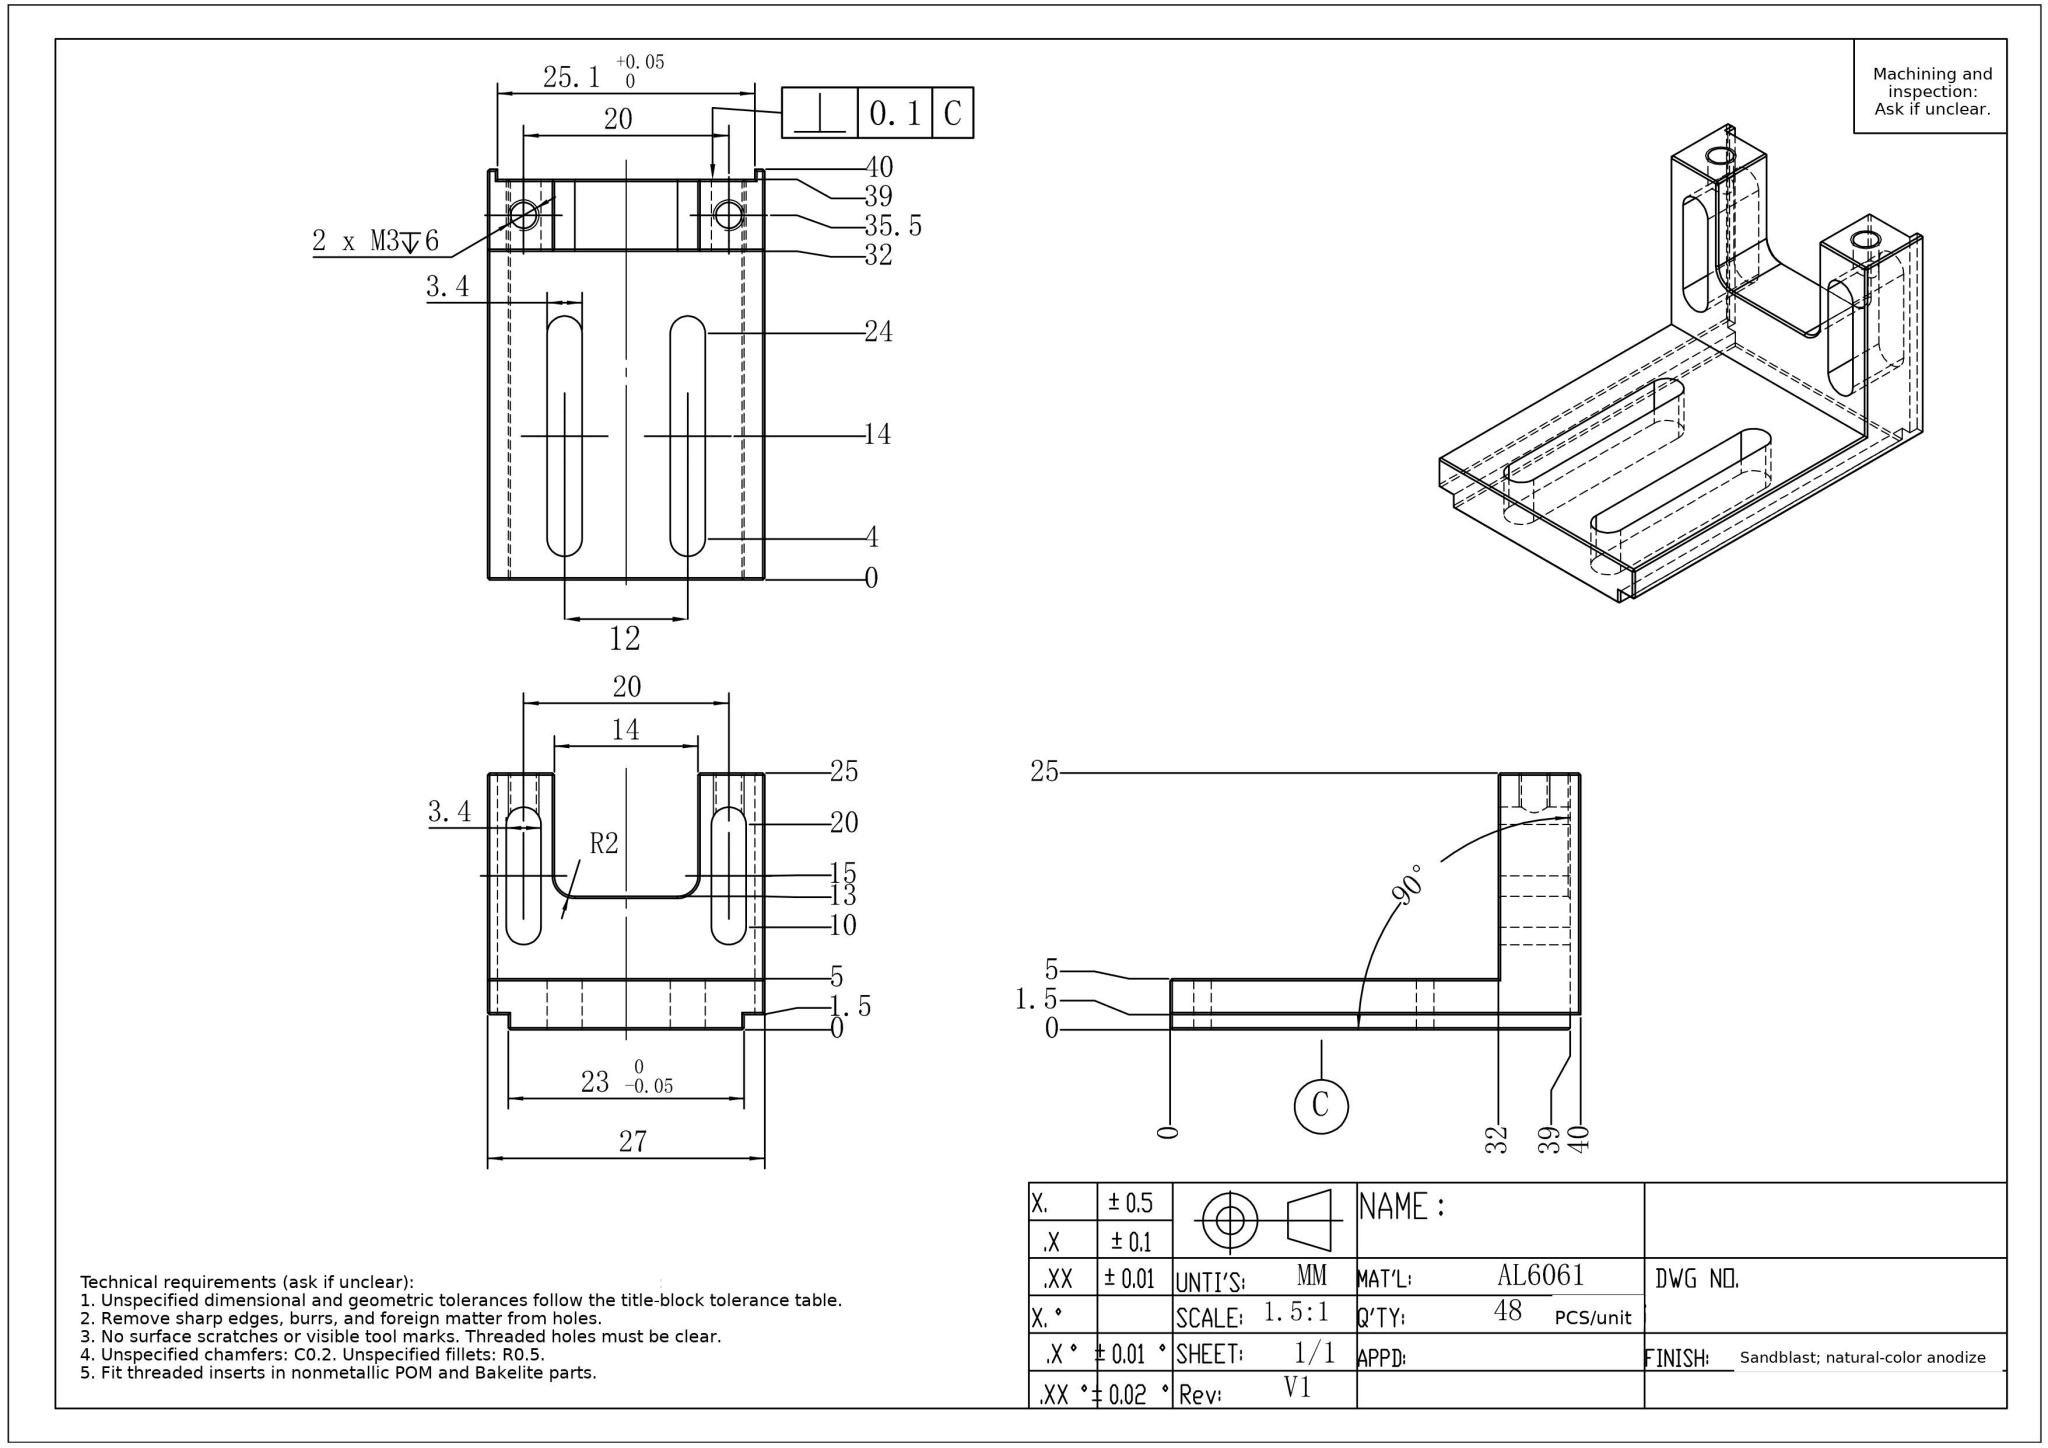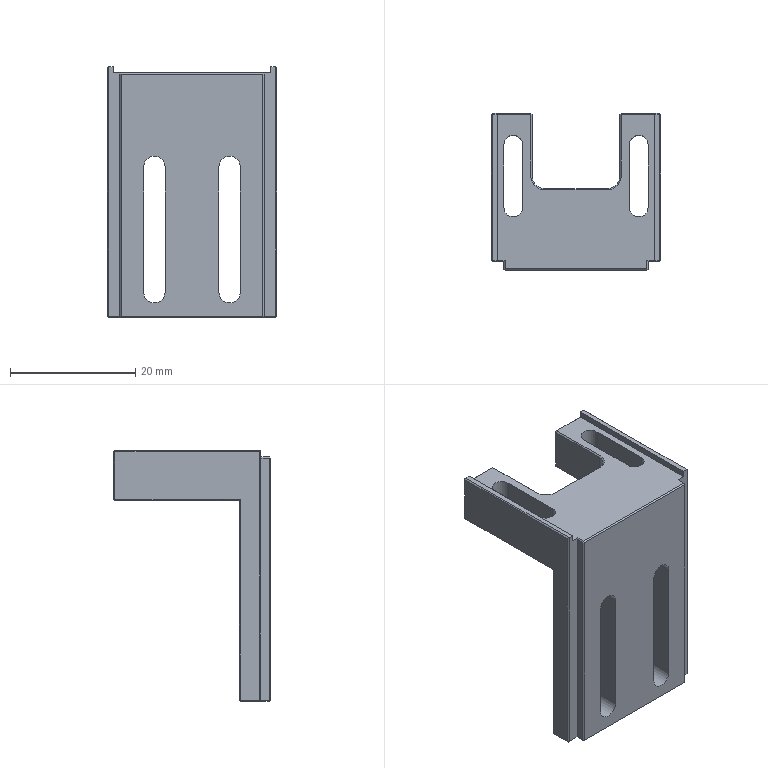Part | NX | mm | 1 solid | 93 faces | box 27 x 25 x 40 mm | volume 6359 mm3 | plane 77 | cylinder 12 | cone 4 | commonest cylinder face diameters 3 x4 3.4 x4 2.4 x2 4 x2